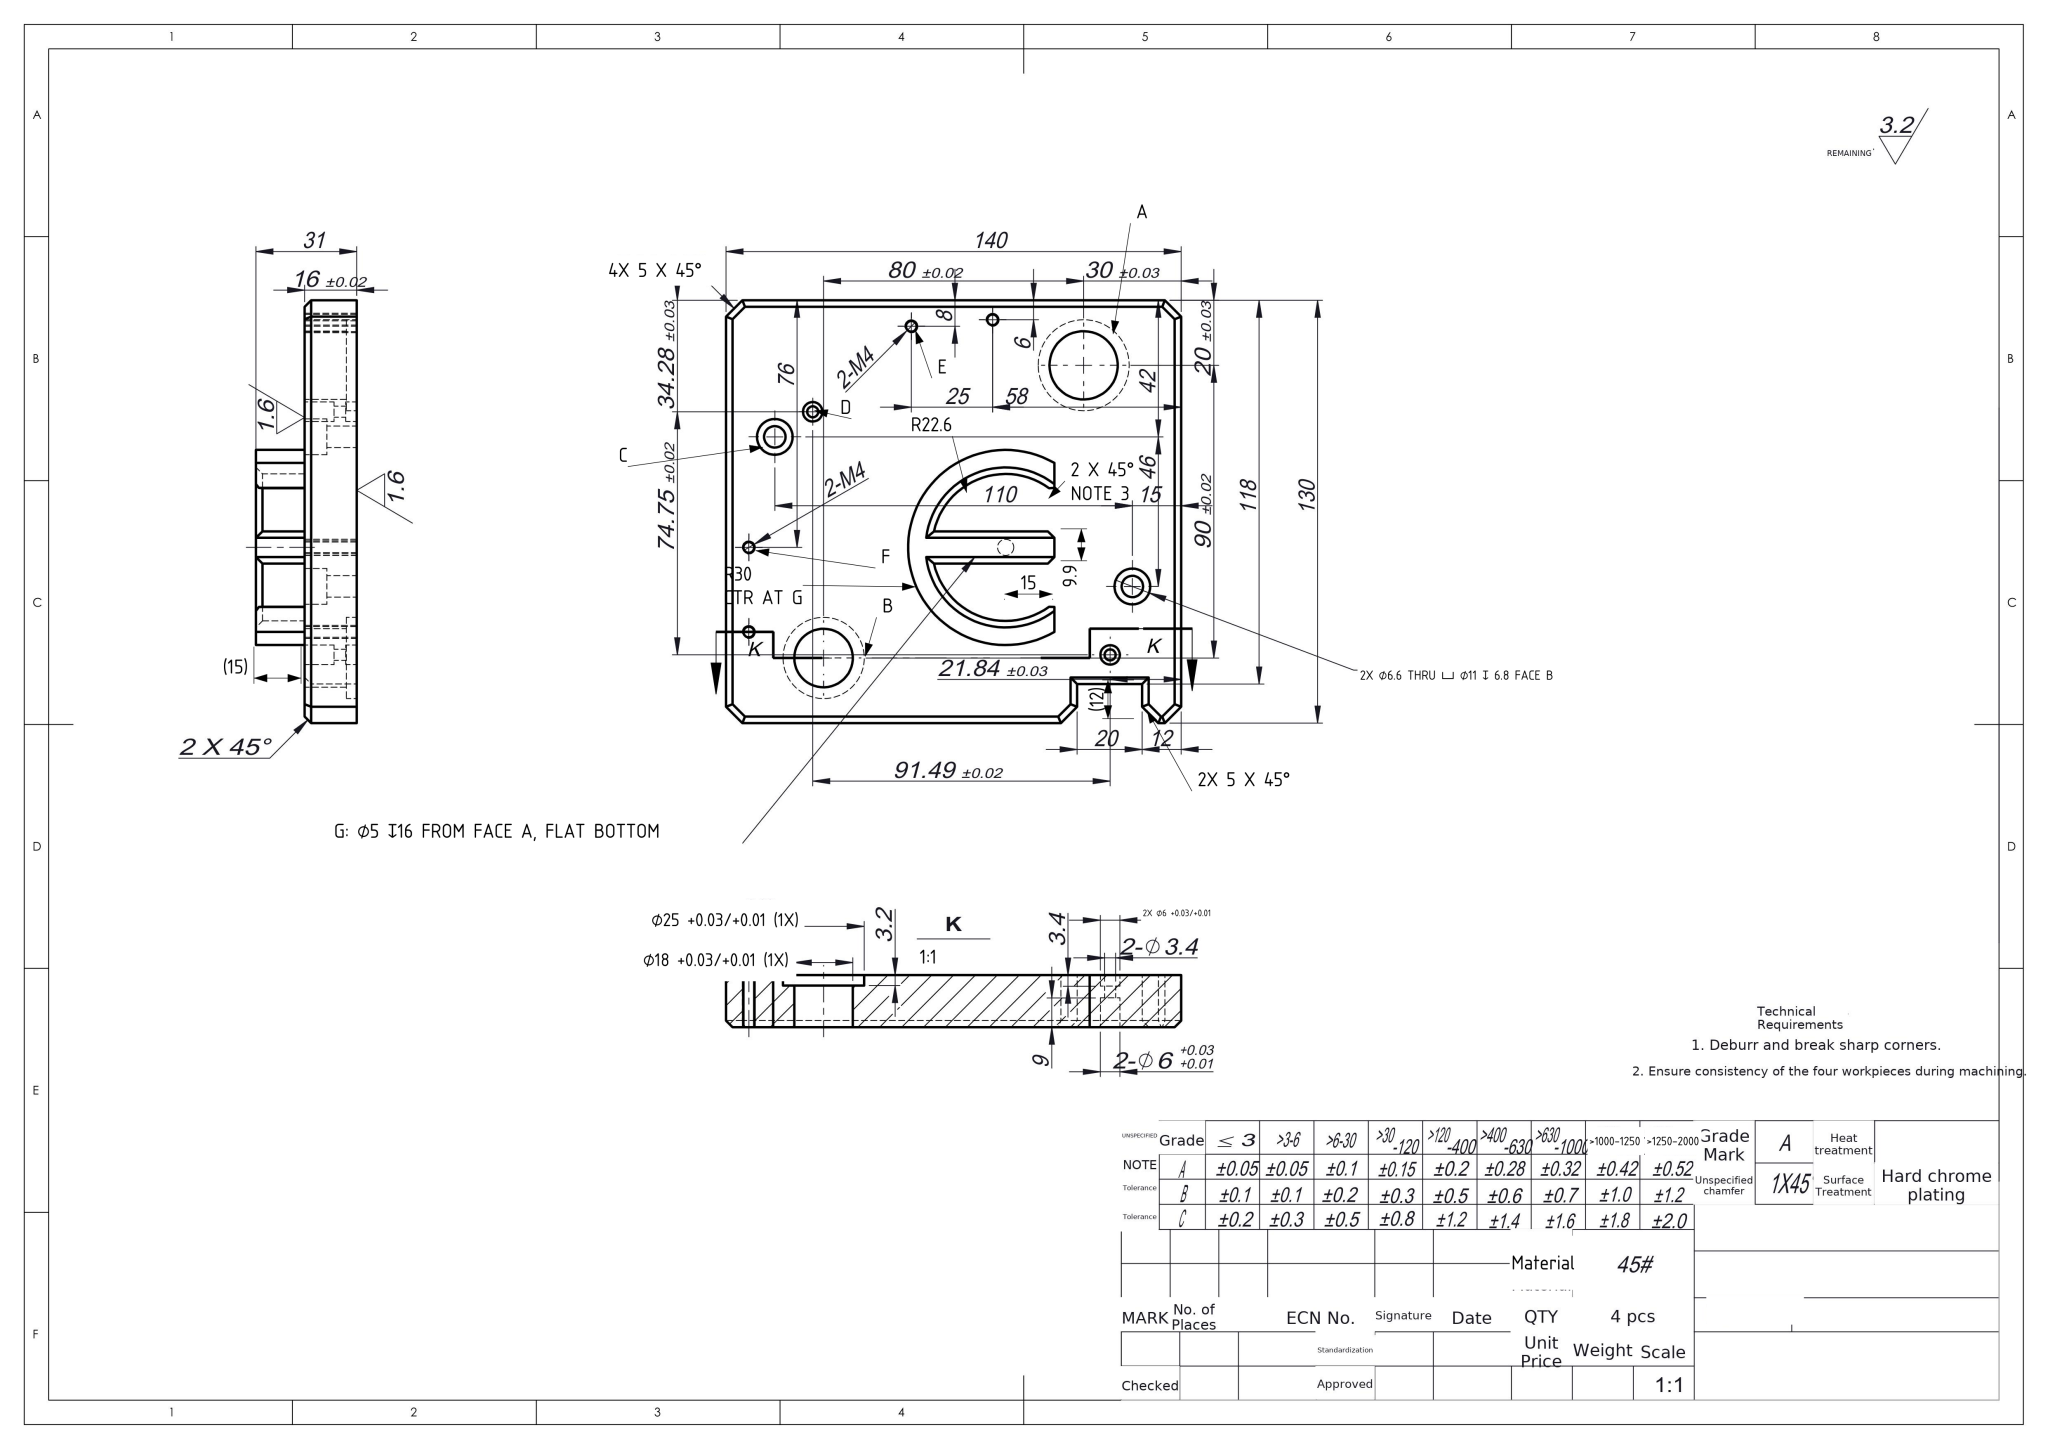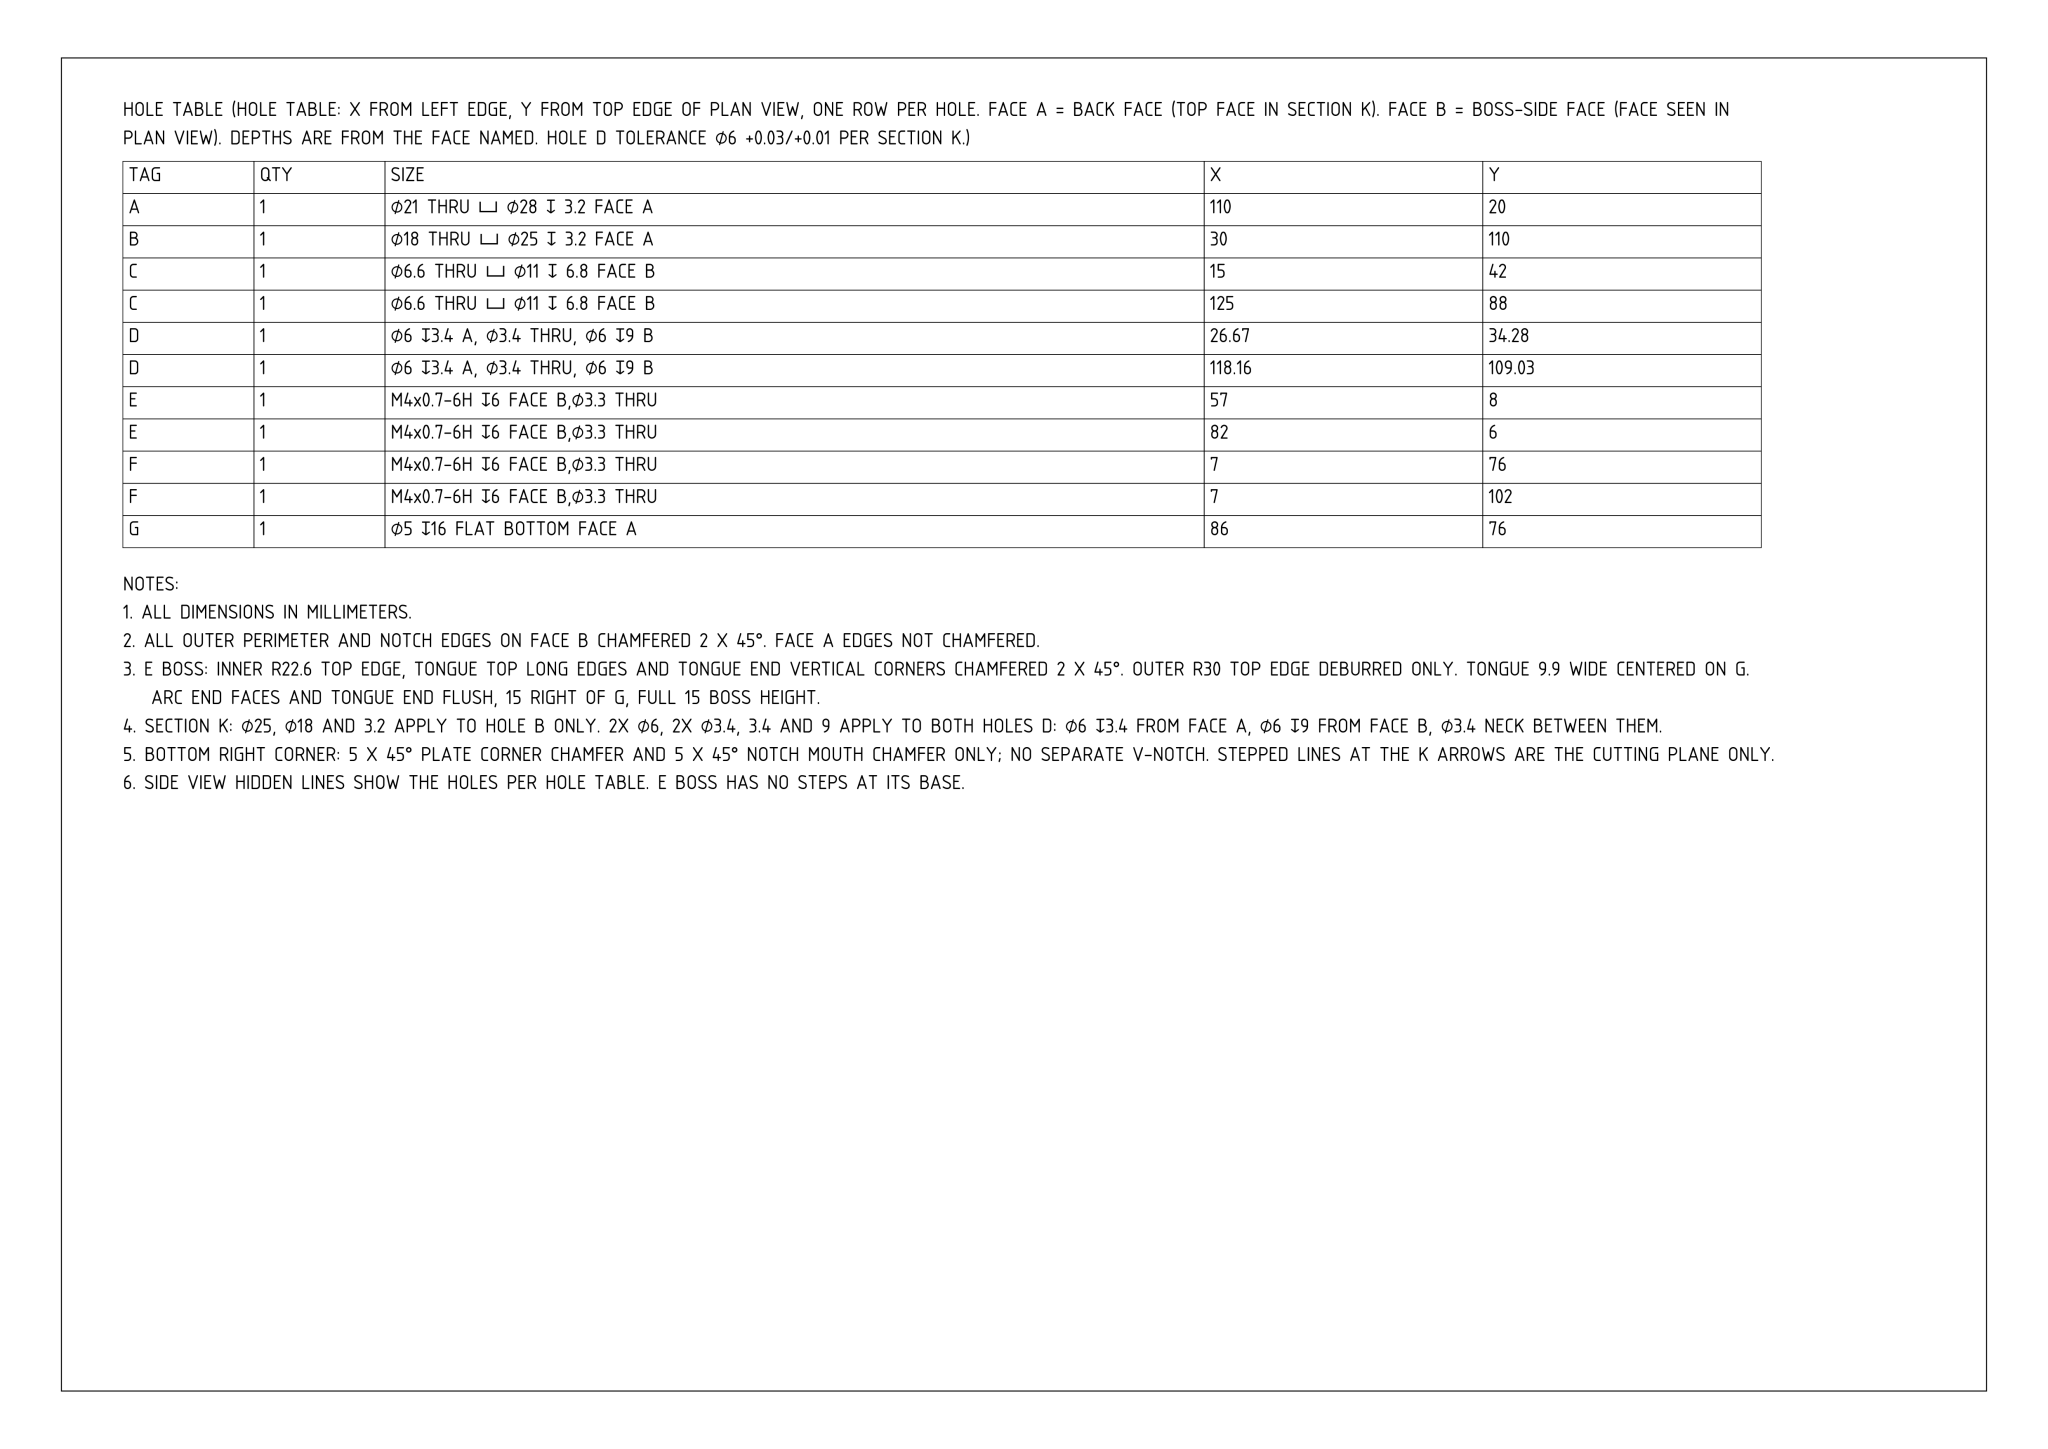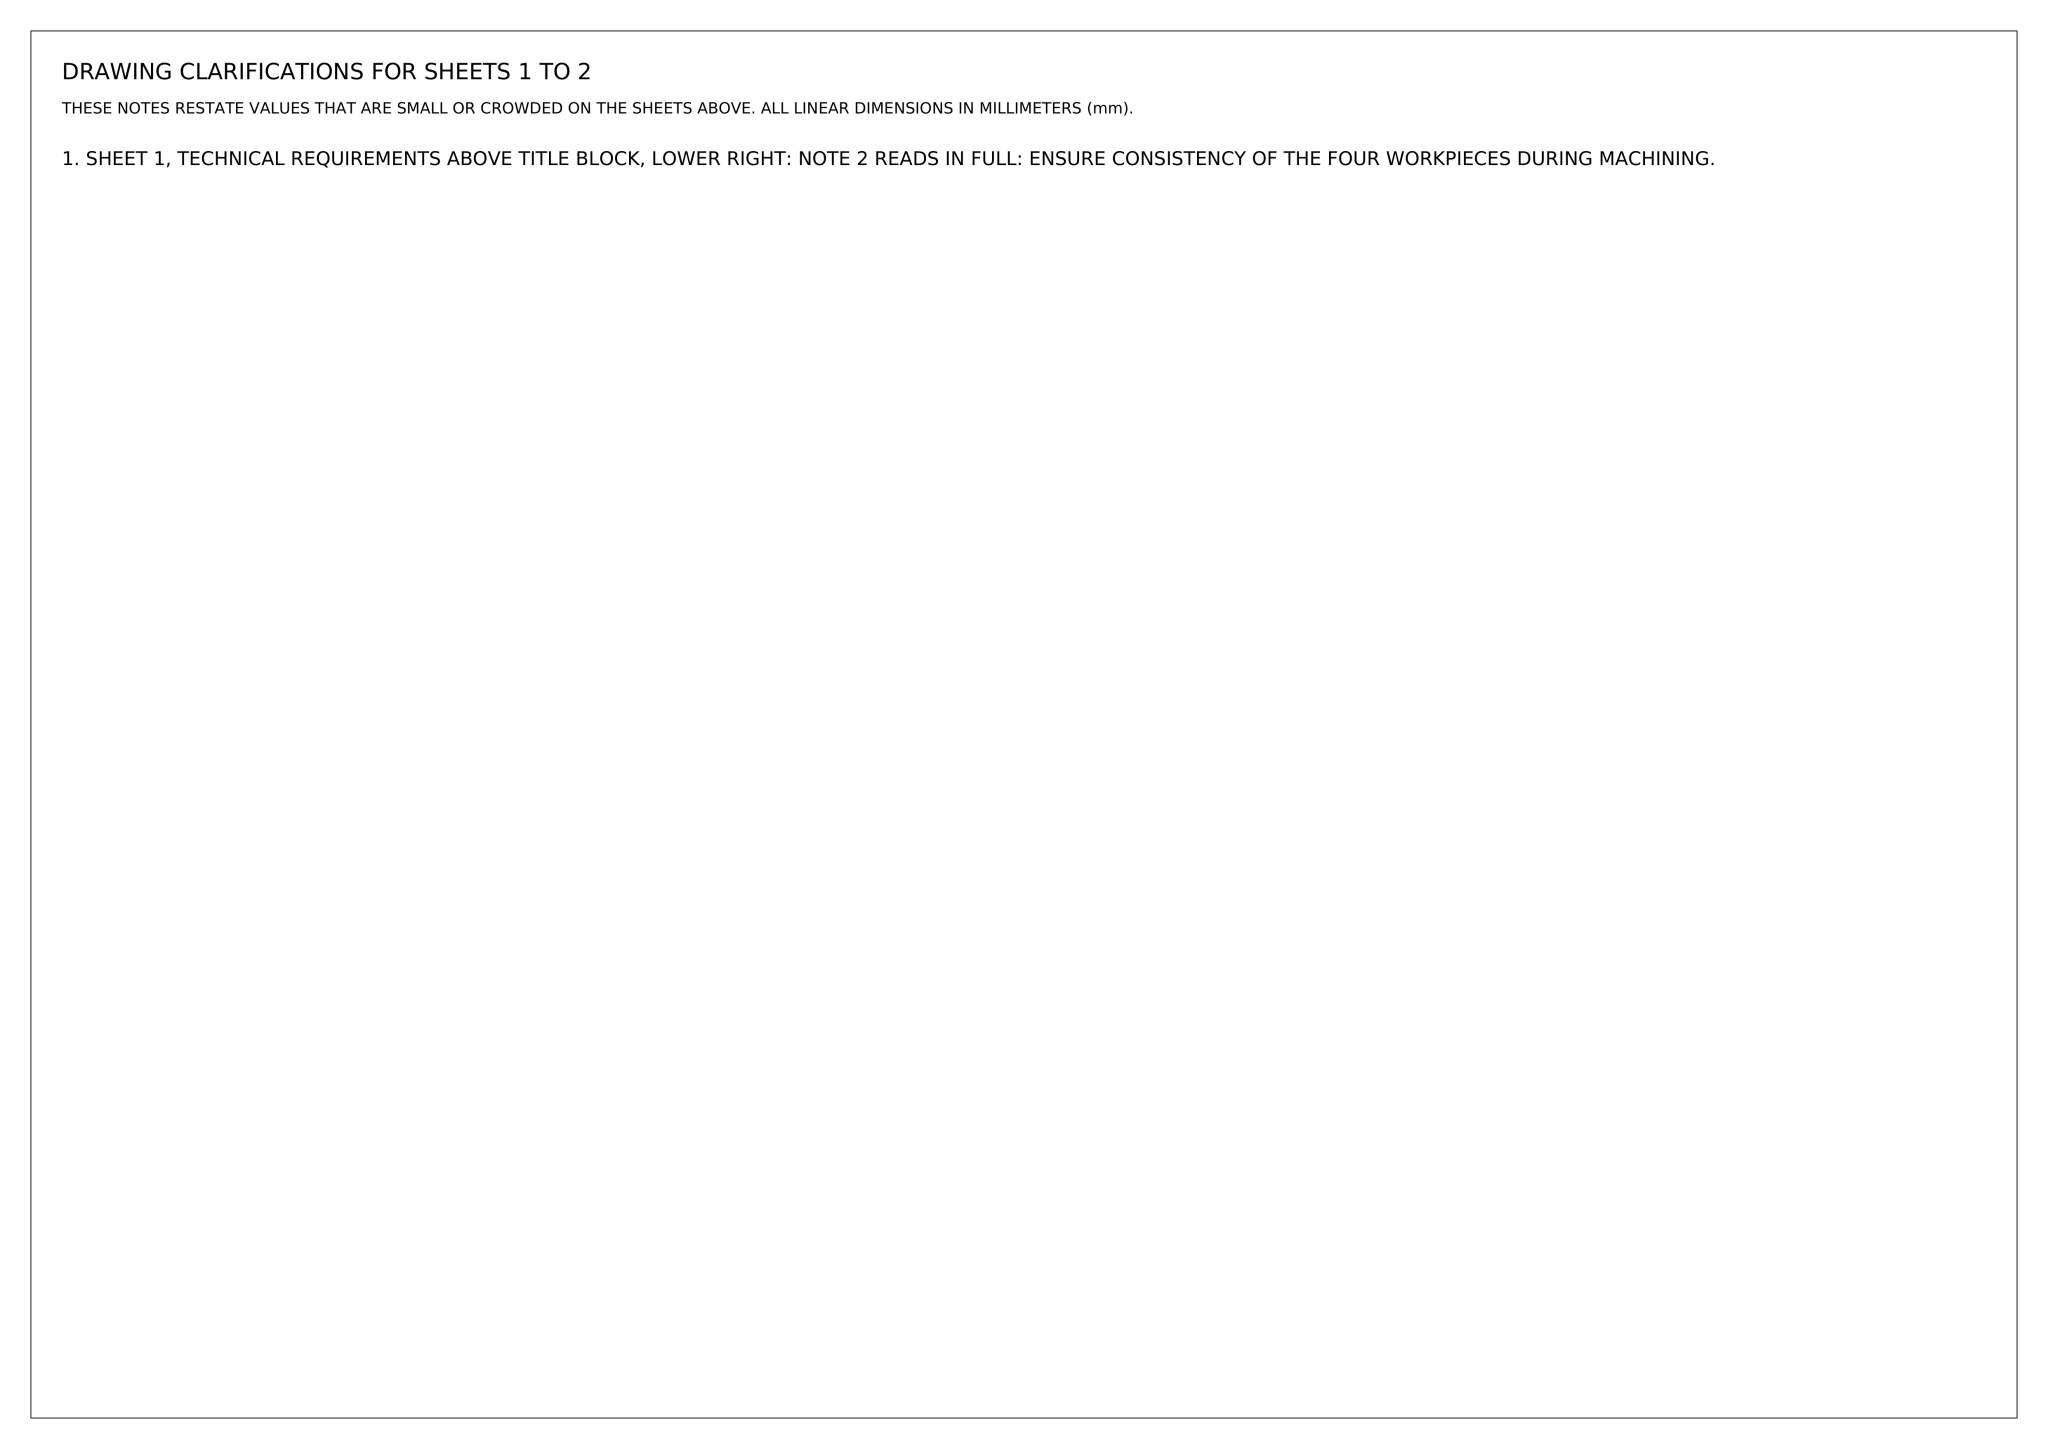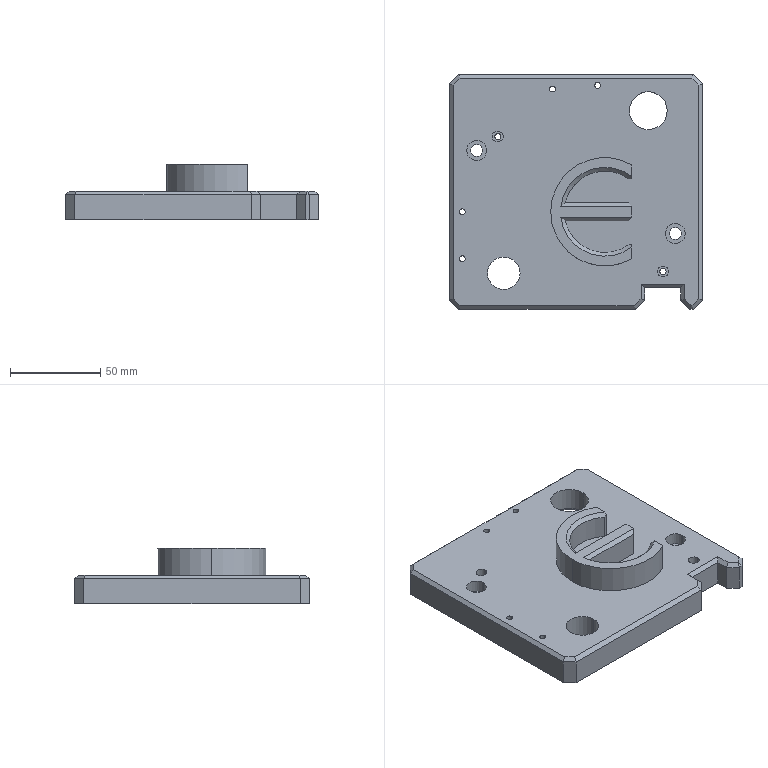Part | NX | mm | 1 solid | 95 faces | box 140 x 130 x 31 mm | volume 288141 mm3 | plane 51 | cylinder 42 | cone 2 | commonest cylinder face diameters 6 x8 3.3 x8 11 x4 6.6 x4 3.4 x4 60 x2 5 x2 28 x2